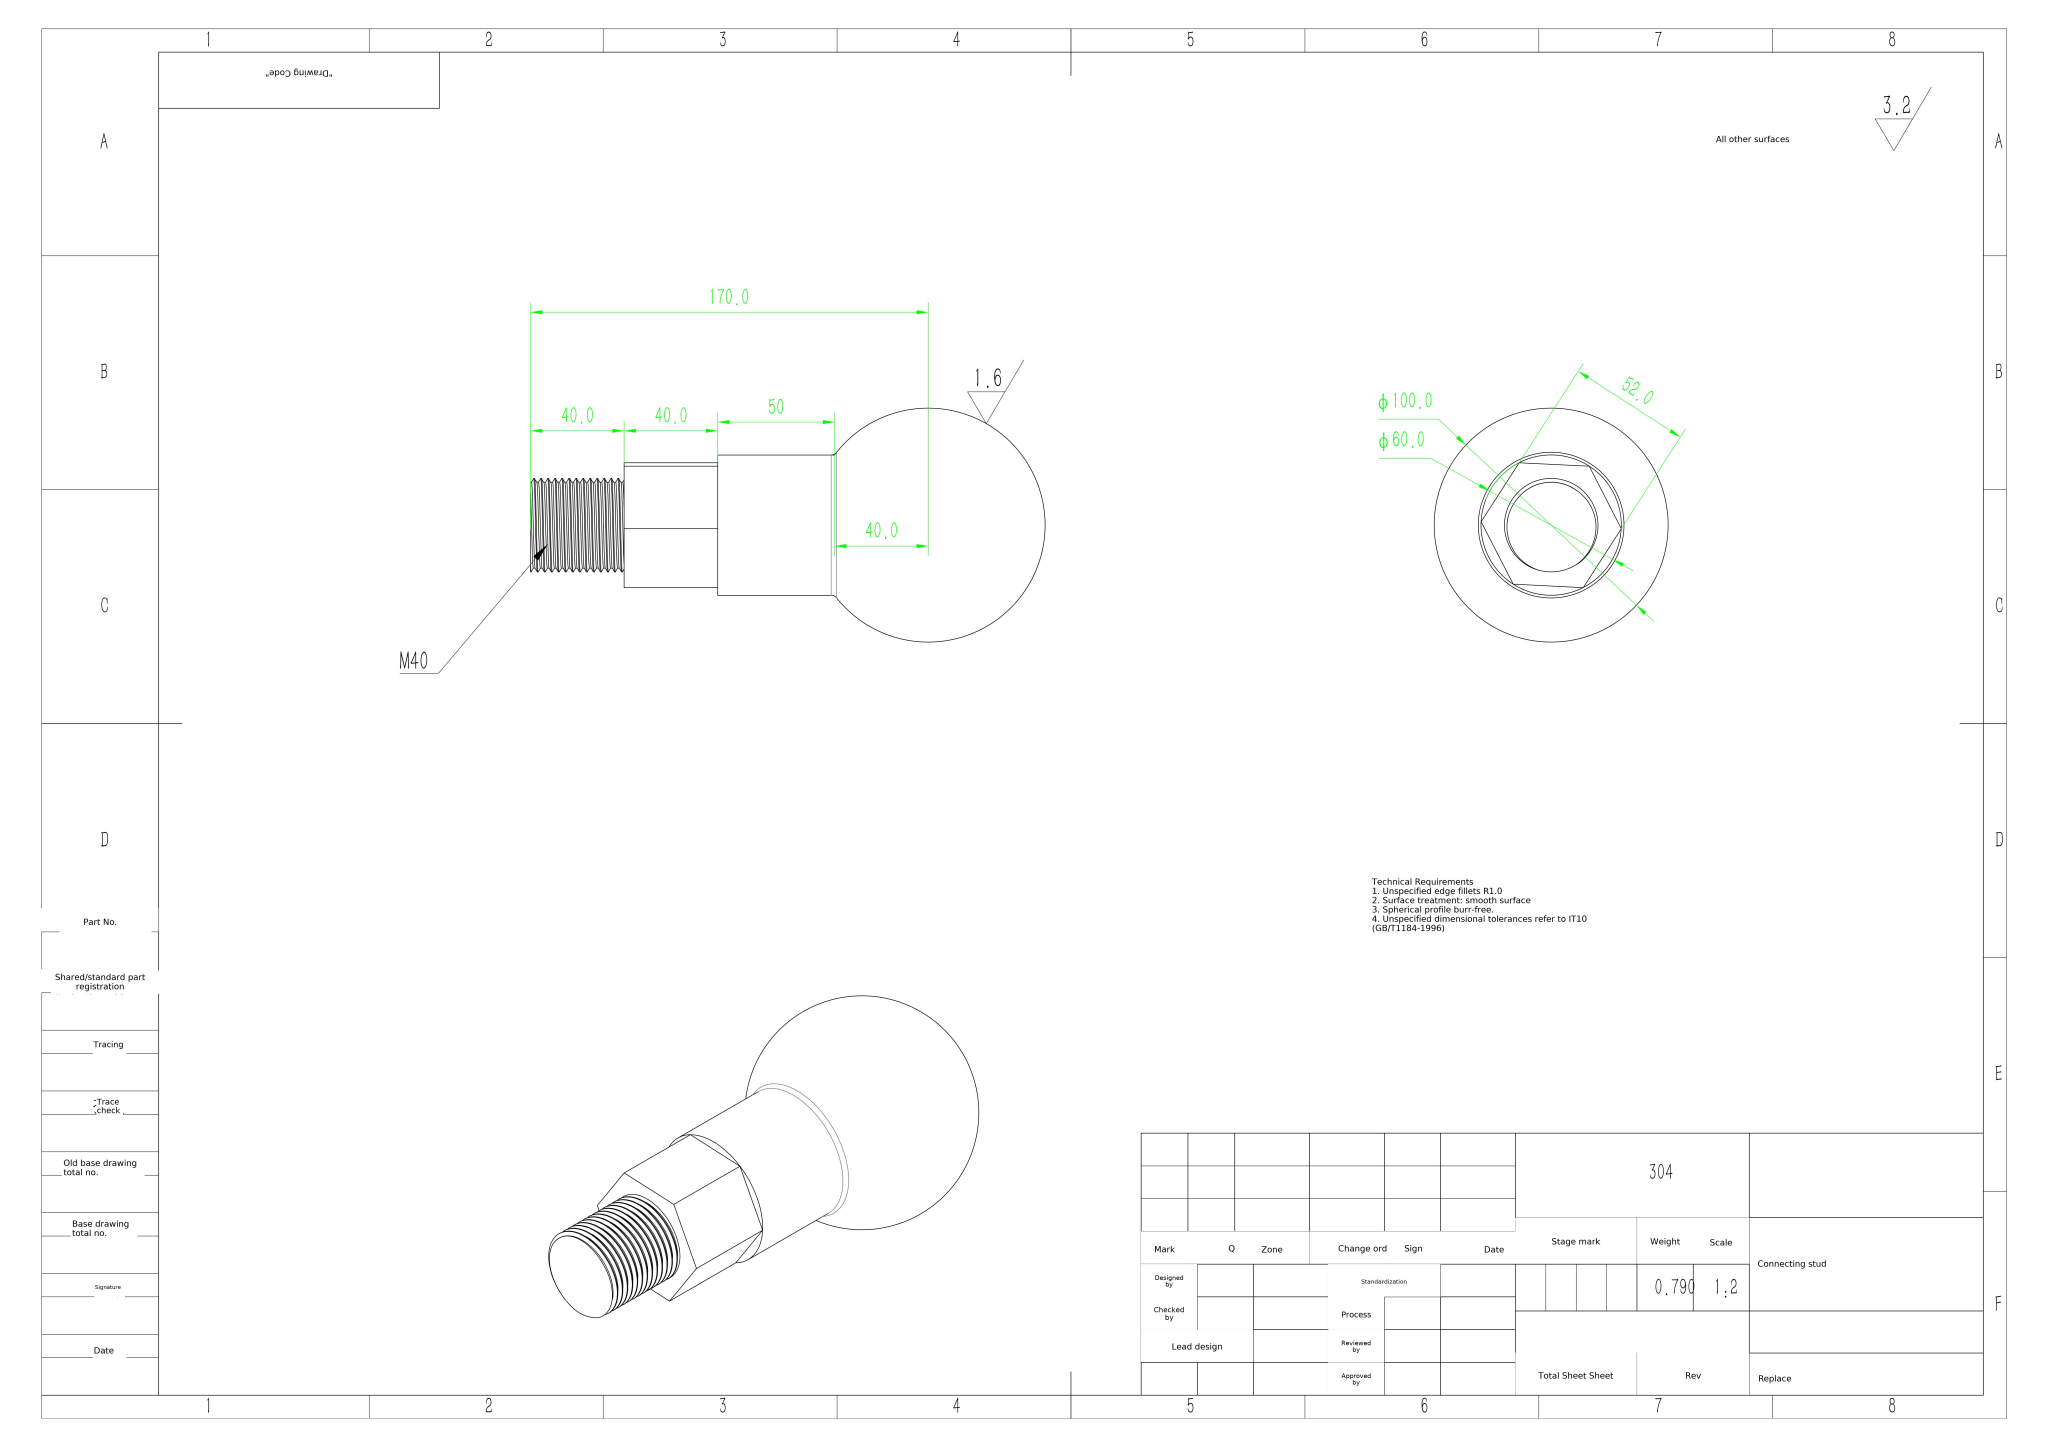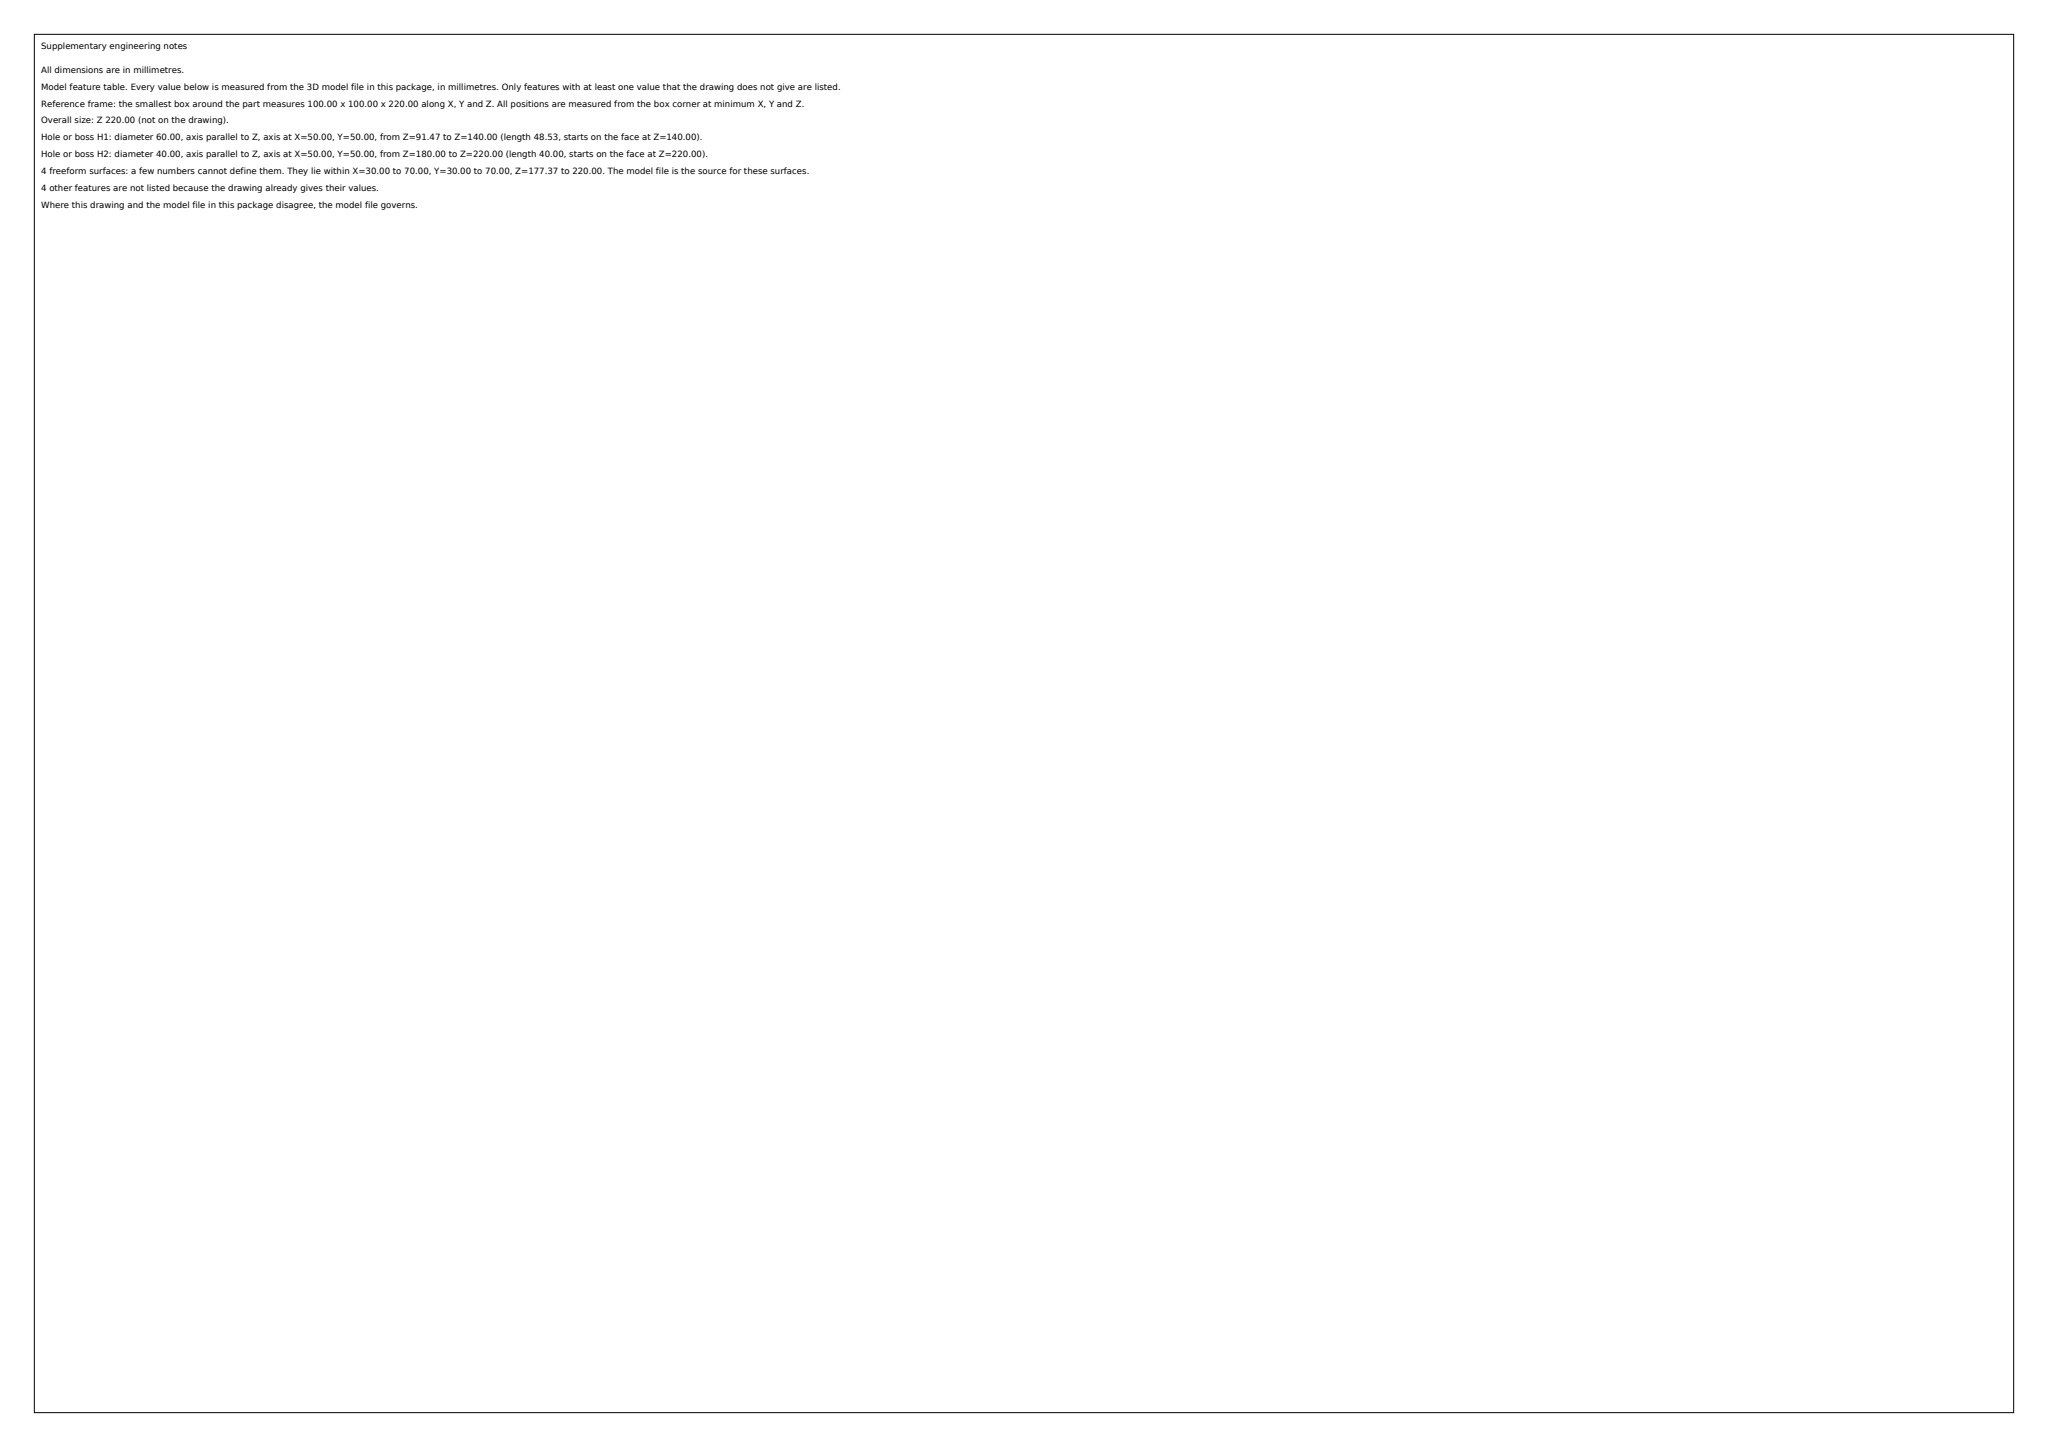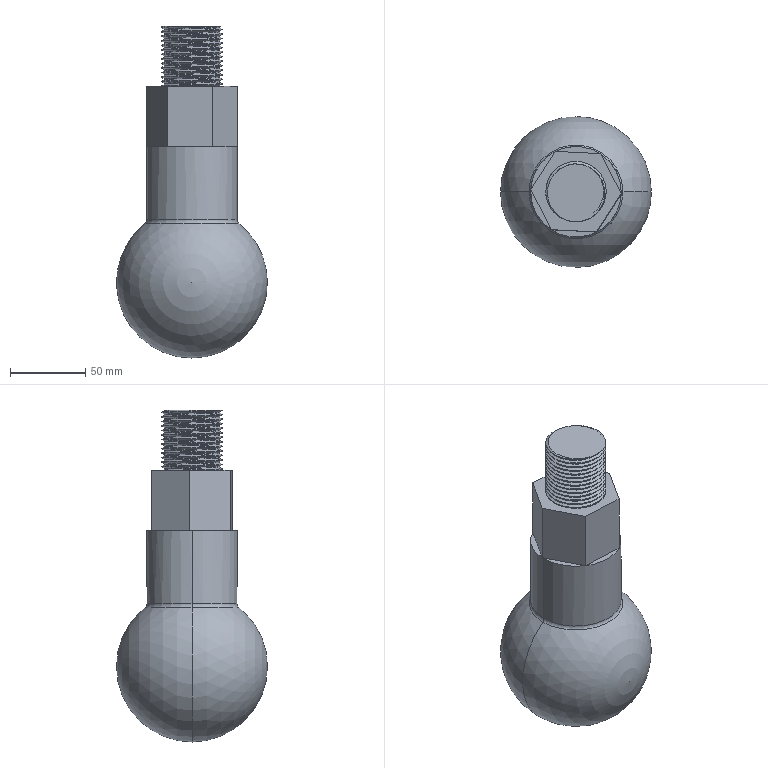Part | SolidWorks | mm | material 304 | 1 solid | 53 faces | box 100 x 100 x 220 mm | volume 789597 mm3 | cylinder 30 | plane 15 | spline 4 | torus 2 | sphere 2 | commonest cylinder face diameters 40 x28 60 x2